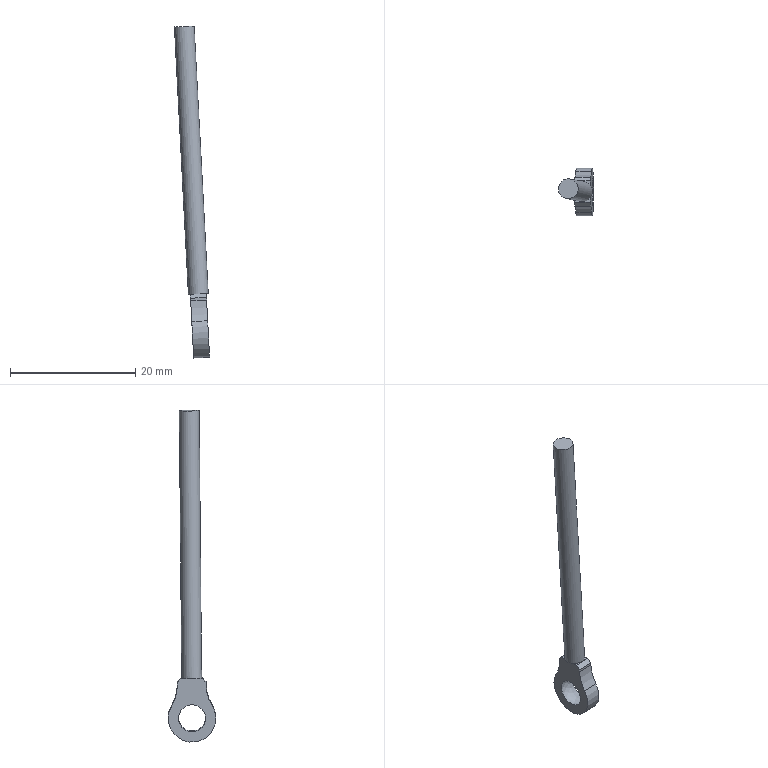Component | NX | TELESCOPIC_ROD_1 | 1 solid | 16 faces | volume 443 mm3 | plane 11 | cylinder 4 | sphere 1 | commonest cylinder face diameters 12.7 x2 7.62 x1 3.175 x1